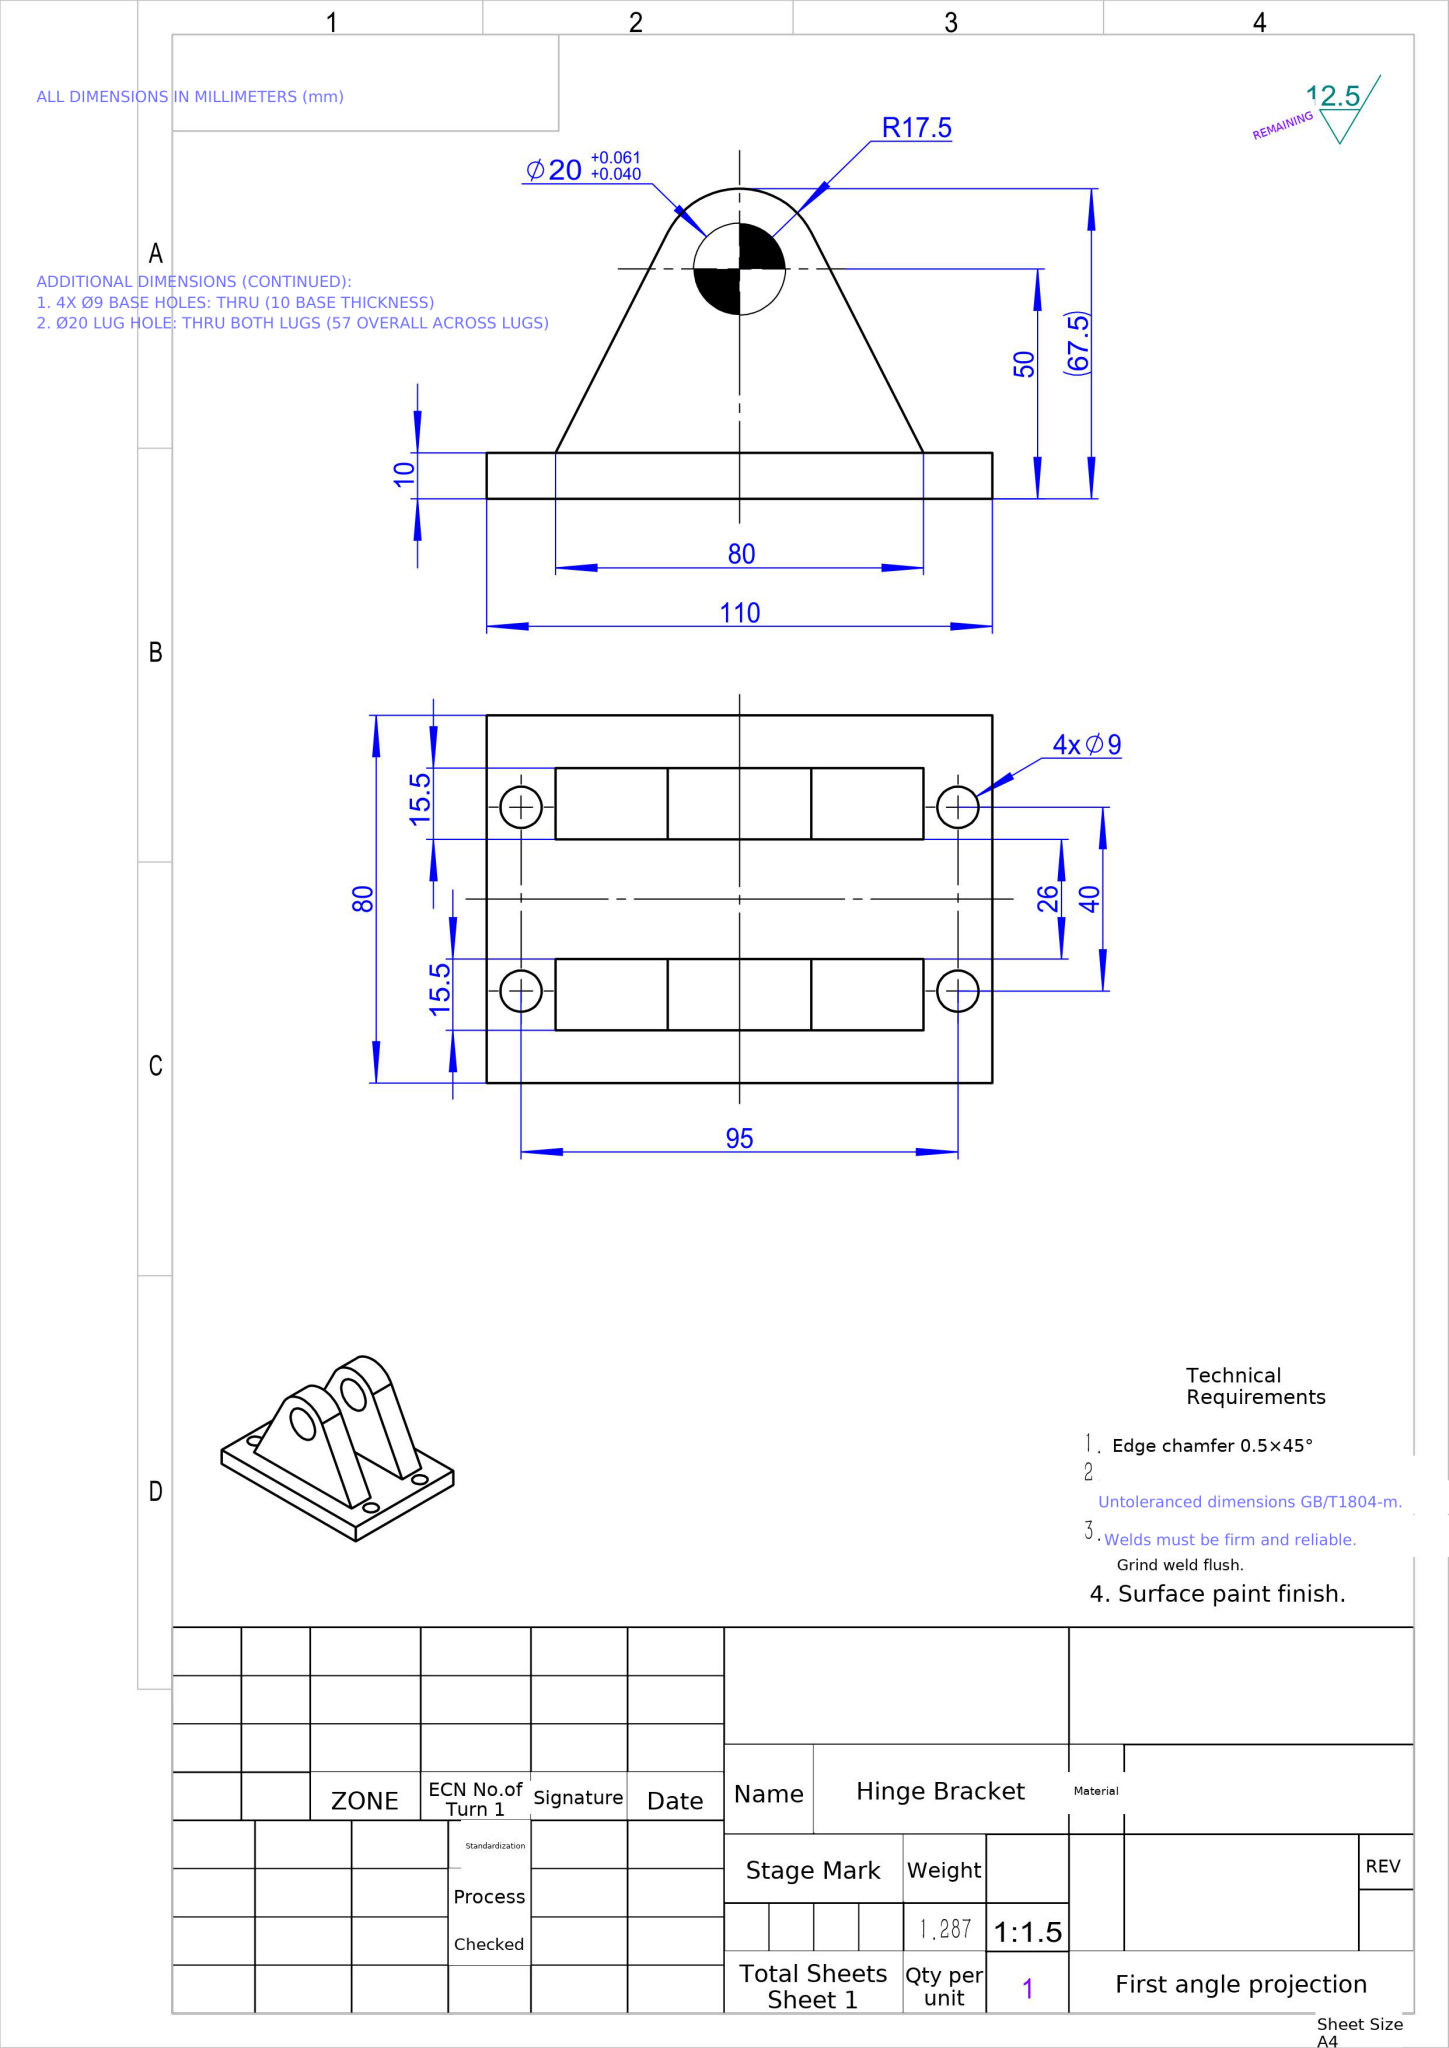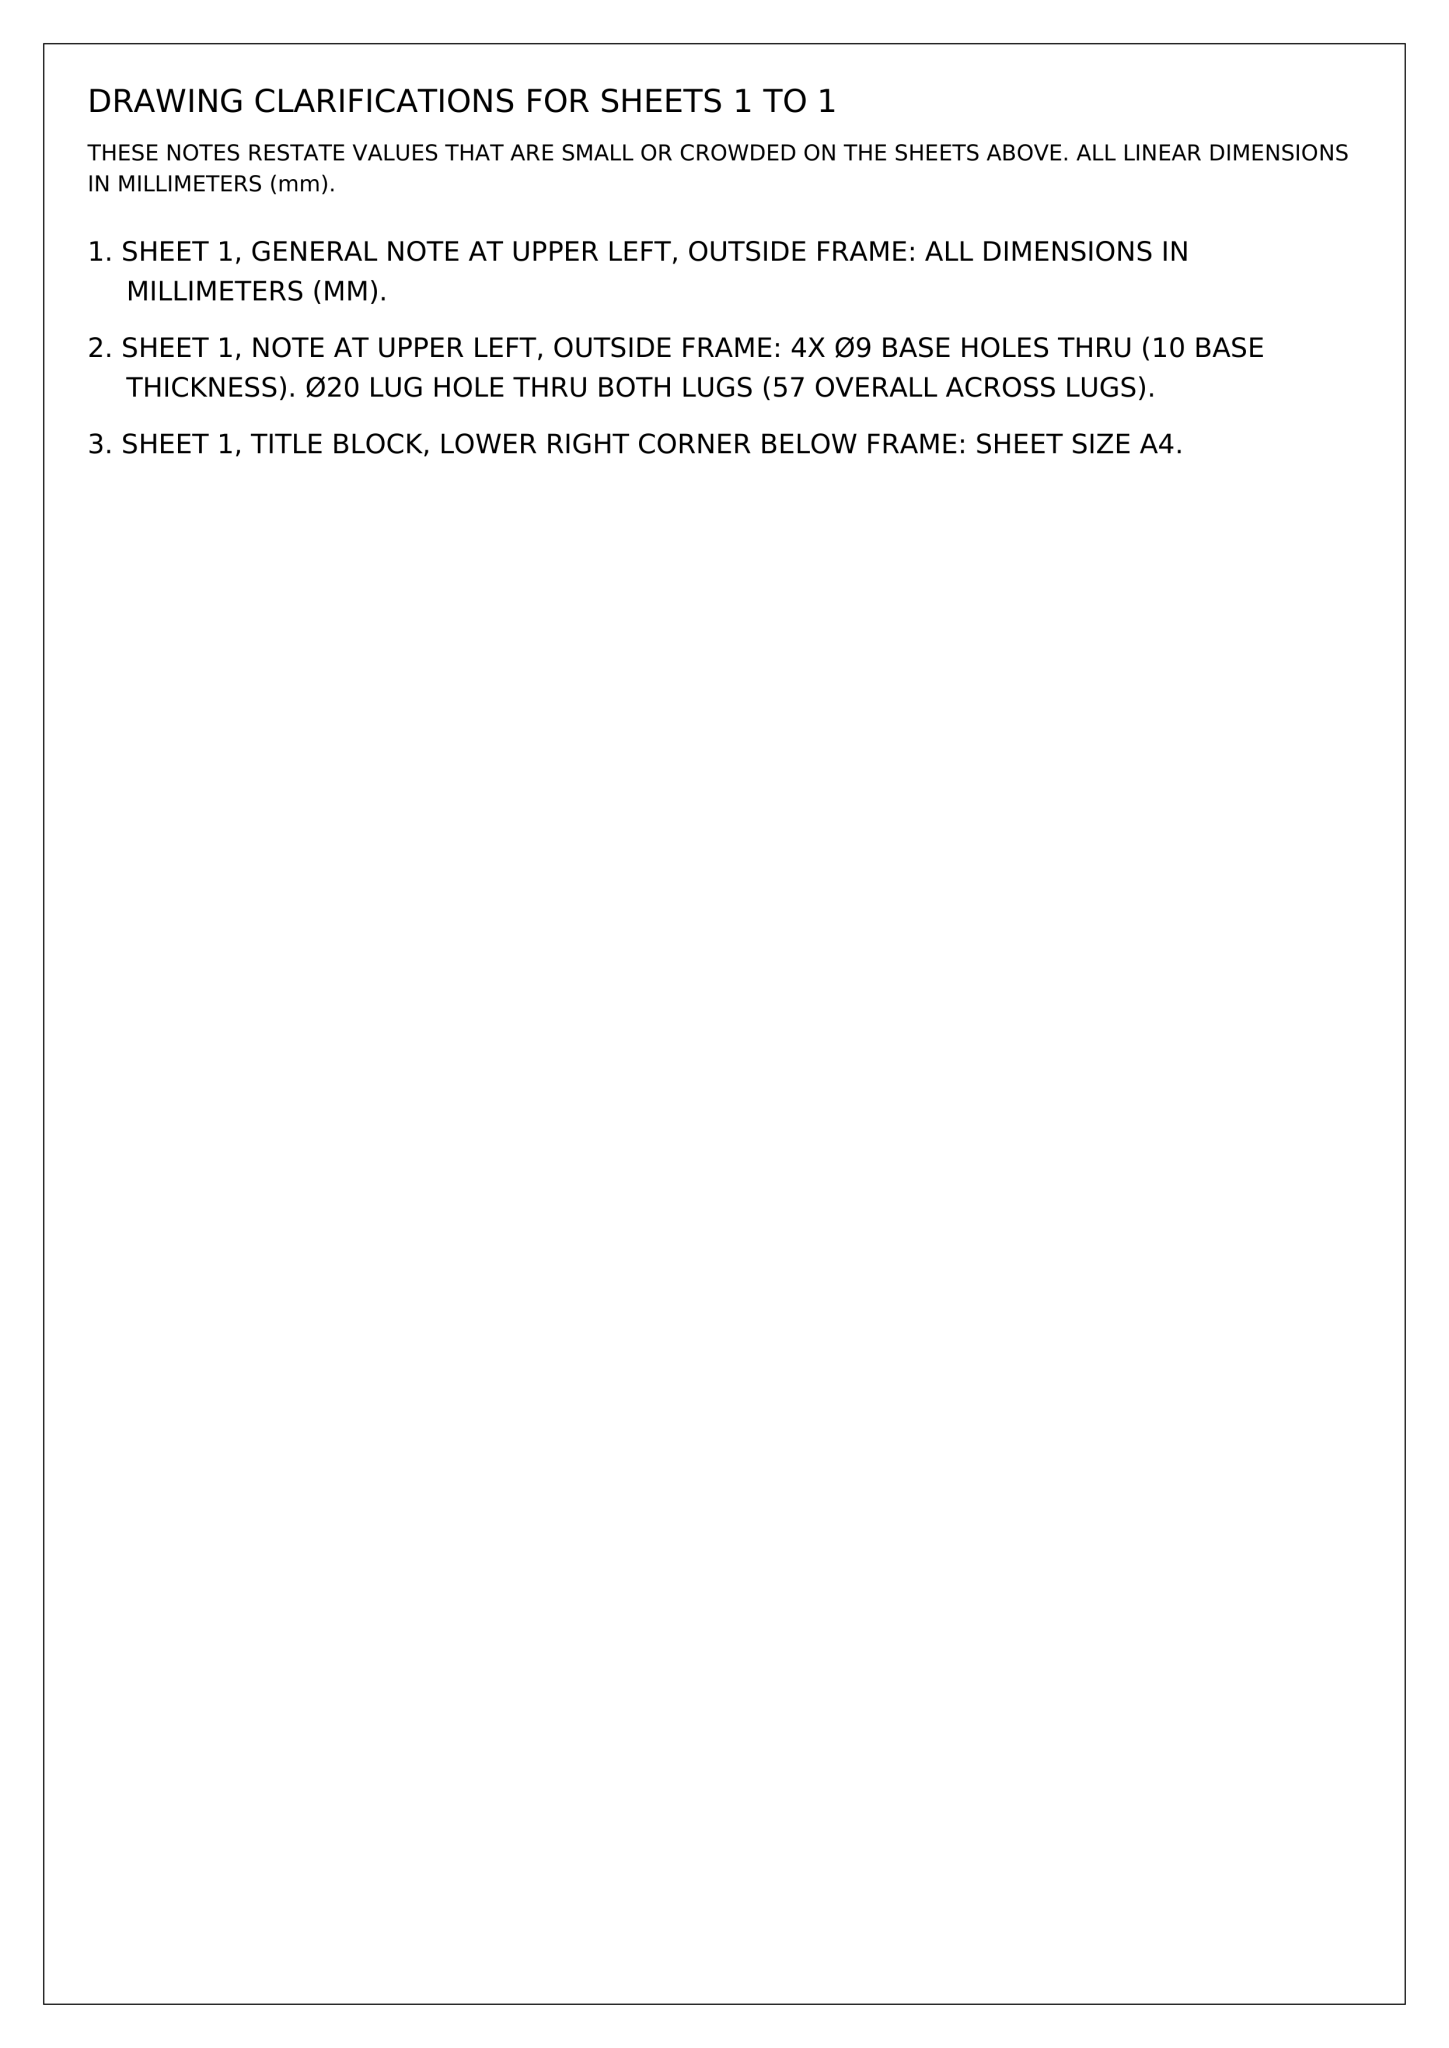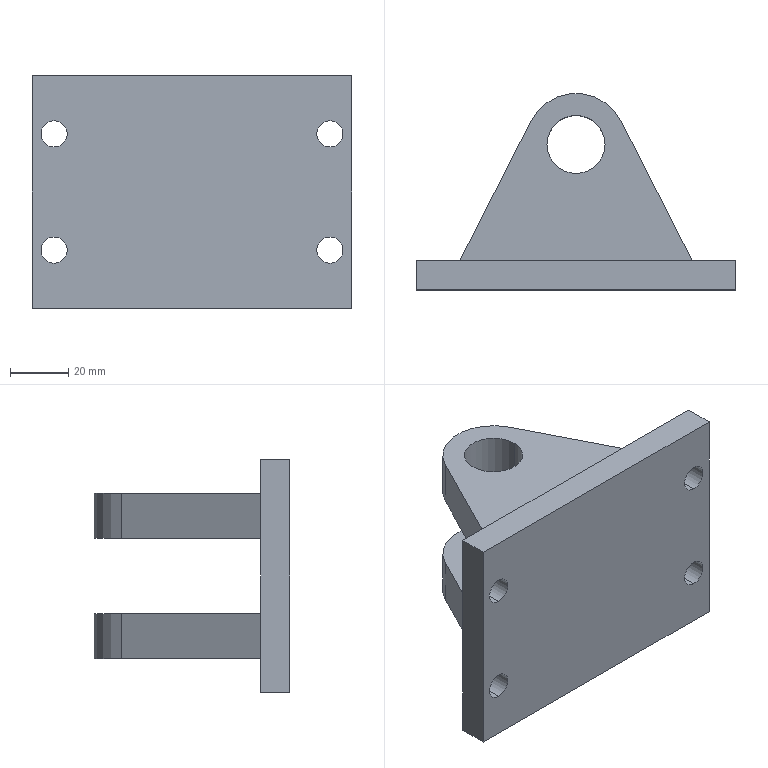Part | NX | mm | 1 solid | 28 faces | box 110 x 67.5 x 80 mm | volume 164942 mm3 | cylinder 14 | plane 14 | commonest cylinder face diameters 9 x8 20 x4 35 x2
STEP:
#1=CARTESIAN_POINT('',(10.,50.,28.5));
#2=VERTEX_POINT('',#1);
#3=CARTESIAN_POINT('',(10.,50.,13.));
#4=VERTEX_POINT('',#3);
#5=CARTESIAN_POINT('',(10.,50.,28.5));
#6=DIRECTION('',(0.,0.,-1.));
#7=VECTOR('',#6,1000.);
#8=LINE('',#5,#7);
#9=EDGE_CURVE('',#2,#4,#8,.T.);
#10=ORIENTED_EDGE('',*,*,#9,.F.);
#11=CARTESIAN_POINT('',(-10.,50.,28.5));
#12=VERTEX_POINT('',#11);
#13=CARTESIAN_POINT('',(0.,50.,28.5));
#14=DIRECTION('',(0.,0.,1.));
#15=DIRECTION('',(1.,0.,0.));
#16=AXIS2_PLACEMENT_3D('',#13,#14,#15);
#17=CIRCLE('',#16,10.);
#18=EDGE_CURVE('',#2,#12,#17,.T.);
#19=ORIENTED_EDGE('',*,*,#18,.T.);
#20=CARTESIAN_POINT('',(-10.,50.,13.));
#21=VERTEX_POINT('',#20);
#22=CARTESIAN_POINT('',(-10.,50.,28.5));
#23=DIRECTION('',(0.,0.,-1.));
#24=VECTOR('',#23,1000.);
#25=LINE('',#22,#24);
#26=EDGE_CURVE('',#12,#21,#25,.T.);
#27=ORIENTED_EDGE('',*,*,#26,.T.);
#28=CARTESIAN_POINT('',(0.,50.,13.));
#29=DIRECTION('',(0.,0.,1.));
#30=DIRECTION('',(1.,0.,0.));
#31=AXIS2_PLACEMENT_3D('',#28,#29,#30);
#32=CIRCLE('',#31,10.);
#33=EDGE_CURVE('',#4,#21,#32,.T.);
#34=ORIENTED_EDGE('',*,*,#33,.F.);
#35=EDGE_LOOP('',(#10,#19,#27,#34));
#36=FACE_OUTER_BOUND('',#35,.T.);
#37=CARTESIAN_POINT('',(0.,50.,28.5));
#38=DIRECTION('',(0.,0.,-1.));
#39=DIRECTION('',(-1.,0.,0.));
#40=AXIS2_PLACEMENT_3D('',#37,#38,#39);
#41=CYLINDRICAL_SURFACE('',#40,10.);
#42=ADVANCED_FACE('',(#36),#41,.F.);
#43=CARTESIAN_POINT('',(-15.595,57.939,13.));
#44=VERTEX_POINT('',#43);
#45=CARTESIAN_POINT('',(-40.,10.,13.));
#46=VERTEX_POINT('',#45);
#47=CARTESIAN_POINT('',(-40.,10.,13.));
#48=DIRECTION('',(-0.4537,-0.8912,0.));
#49=VECTOR('',#48,1000.);
#50=LINE('',#47,#49);
#51=EDGE_CURVE('',#44,#46,#50,.T.);
#52=ORIENTED_EDGE('',*,*,#51,.T.);
#53=CARTESIAN_POINT('',(-40.,10.,28.5));
#54=VERTEX_POINT('',#53);
#55=CARTESIAN_POINT('',(-40.,10.,28.5));
#56=DIRECTION('',(0.,0.,-1.));
#57=VECTOR('',#56,1000.);
#58=LINE('',#55,#57);
#59=EDGE_CURVE('',#54,#46,#58,.T.);
#60=ORIENTED_EDGE('',*,*,#59,.F.);
#61=CARTESIAN_POINT('',(-15.595,57.939,28.5));
#62=VERTEX_POINT('',#61);
#63=CARTESIAN_POINT('',(-40.,10.,28.5));
#64=DIRECTION('',(-0.4537,-0.8912,0.));
#65=VECTOR('',#64,1000.);
#66=LINE('',#63,#65);
#67=EDGE_CURVE('',#62,#54,#66,.T.);
#68=ORIENTED_EDGE('',*,*,#67,.F.);
#69=CARTESIAN_POINT('',(-15.595,57.939,28.5));
#70=DIRECTION('',(0.,0.,-1.));
#71=VECTOR('',#70,1000.);
#72=LINE('',#69,#71);
#73=EDGE_CURVE('',#62,#44,#72,.T.);
#74=ORIENTED_EDGE('',*,*,#73,.T.);
#75=EDGE_LOOP('',(#52,#60,#68,#74));
#76=FACE_OUTER_BOUND('',#75,.T.);
#77=CARTESIAN_POINT('',(-40.,10.,28.5));
#78=DIRECTION('',(0.8912,-0.4537,0.));
#79=DIRECTION('',(0.,0.,-1.));
#80=AXIS2_PLACEMENT_3D('',#77,#78,#79);
#81=PLANE('',#80);
#82=ADVANCED_FACE('',(#76),#81,.F.);
#83=CARTESIAN_POINT('',(15.595,57.939,13.));
#84=VERTEX_POINT('',#83);
#85=CARTESIAN_POINT('',(0.,50.,13.));
#86=DIRECTION('',(0.,0.,1.));
#87=DIRECTION('',(1.,0.,0.));
#88=AXIS2_PLACEMENT_3D('',#85,#86,#87);
#89=CIRCLE('',#88,17.5);
#90=EDGE_CURVE('',#84,#44,#89,.T.);
#91=ORIENTED_EDGE('',*,*,#90,.T.);
#92=ORIENTED_EDGE('',*,*,#73,.F.);
#93=CARTESIAN_POINT('',(15.595,57.939,28.5));
#94=VERTEX_POINT('',#93);
#95=CARTESIAN_POINT('',(0.,50.,28.5));
#96=DIRECTION('',(0.,0.,1.));
#97=DIRECTION('',(1.,0.,0.));
#98=AXIS2_PLACEMENT_3D('',#95,#96,#97);
#99=CIRCLE('',#98,17.5);
#100=EDGE_CURVE('',#94,#62,#99,.T.);
#101=ORIENTED_EDGE('',*,*,#100,.F.);
#102=CARTESIAN_POINT('',(15.595,57.939,28.5));
#103=DIRECTION('',(0.,0.,-1.));
#104=VECTOR('',#103,1000.);
#105=LINE('',#102,#104);
#106=EDGE_CURVE('',#94,#84,#105,.T.);
#107=ORIENTED_EDGE('',*,*,#106,.T.);
#108=EDGE_LOOP('',(#91,#92,#101,#107));
#109=FACE_OUTER_BOUND('',#108,.T.);
#110=CARTESIAN_POINT('',(0.,50.,28.5));
#111=DIRECTION('',(0.,0.,-1.));
#112=DIRECTION('',(-1.,0.,0.));
#113=AXIS2_PLACEMENT_3D('',#110,#111,#112);
#114=CYLINDRICAL_SURFACE('',#113,17.5);
#115=ADVANCED_FACE('',(#109),#114,.T.);
#116=CARTESIAN_POINT('',(40.,10.,13.));
#117=VERTEX_POINT('',#116);
#118=CARTESIAN_POINT('',(40.,10.,13.));
#119=DIRECTION('',(-0.4537,0.8912,0.));
#120=VECTOR('',#119,1000.);
#121=LINE('',#118,#120);
#122=EDGE_CURVE('',#117,#84,#121,.T.);
#123=ORIENTED_EDGE('',*,*,#122,.T.);
#124=ORIENTED_EDGE('',*,*,#106,.F.);
#125=CARTESIAN_POINT('',(40.,10.,28.5));
#126=VERTEX_POINT('',#125);
#127=CARTESIAN_POINT('',(40.,10.,28.5));
#128=DIRECTION('',(-0.4537,0.8912,0.));
#129=VECTOR('',#128,1000.);
#130=LINE('',#127,#129);
#131=EDGE_CURVE('',#126,#94,#130,.T.);
#132=ORIENTED_EDGE('',*,*,#131,.F.);
#133=CARTESIAN_POINT('',(40.,10.,28.5));
#134=DIRECTION('',(0.,0.,-1.));
#135=VECTOR('',#134,1000.);
#136=LINE('',#133,#135);
#137=EDGE_CURVE('',#126,#117,#136,.T.);
#138=ORIENTED_EDGE('',*,*,#137,.T.);
#139=EDGE_LOOP('',(#123,#124,#132,#138));
#140=FACE_OUTER_BOUND('',#139,.T.);
#141=CARTESIAN_POINT('',(40.,10.,28.5));
#142=DIRECTION('',(-0.8912,-0.4537,0.));
#143=DIRECTION('',(-0.4537,0.8912,0.));
#144=AXIS2_PLACEMENT_3D('',#141,#142,#143);
#145=PLANE('',#144);
#146=ADVANCED_FACE('',(#140),#145,.F.);
#147=CARTESIAN_POINT('',(0.,50.,13.));
#148=DIRECTION('',(0.,0.,1.));
#149=DIRECTION('',(1.,0.,0.));
#150=AXIS2_PLACEMENT_3D('',#147,#148,#149);
#151=CIRCLE('',#150,10.);
#152=EDGE_CURVE('',#21,#4,#151,.T.);
#153=ORIENTED_EDGE('',*,*,#152,.T.);
#154=ORIENTED_EDGE('',*,*,#33,.T.);
#155=EDGE_LOOP('',(#153,#154));
#156=FACE_BOUND('',#155,.T.);
#157=CARTESIAN_POINT('',(-40.,10.,13.));
#158=DIRECTION('',(1.,0.,0.));
#159=VECTOR('',#158,1000.);
#160=LINE('',#157,#159);
#161=EDGE_CURVE('',#46,#117,#160,.T.);
#162=ORIENTED_EDGE('',*,*,#161,.F.);
#163=ORIENTED_EDGE('',*,*,#51,.F.);
#164=ORIENTED_EDGE('',*,*,#90,.F.);
#165=ORIENTED_EDGE('',*,*,#122,.F.);
#166=EDGE_LOOP('',(#162,#163,#164,#165));
#167=FACE_OUTER_BOUND('',#166,.T.);
#168=CARTESIAN_POINT('',(0.,50.,13.));
#169=DIRECTION('',(0.,0.,1.));
#170=DIRECTION('',(1.,0.,0.));
#171=AXIS2_PLACEMENT_3D('',#168,#169,#170);
#172=PLANE('',#171);
#173=ADVANCED_FACE('',(#156,#167),#172,.F.);
#174=CARTESIAN_POINT('',(0.,50.,28.5));
#175=DIRECTION('',(0.,0.,1.));
#176=DIRECTION('',(1.,0.,0.));
#177=AXIS2_PLACEMENT_3D('',#174,#175,#176);
#178=CIRCLE('',#177,10.);
#179=EDGE_CURVE('',#12,#2,#178,.T.);
#180=ORIENTED_EDGE('',*,*,#179,.F.);
#181=ORIENTED_EDGE('',*,*,#18,.F.);
#182=EDGE_LOOP('',(#180,#181));
#183=FACE_BOUND('',#182,.T.);
#184=CARTESIAN_POINT('',(-40.,10.,28.5));
#185=DIRECTION('',(1.,0.,0.));
#186=VECTOR('',#185,1000.);
#187=LINE('',#184,#186);
#188=EDGE_CURVE('',#54,#126,#187,.T.);
#189=ORIENTED_EDGE('',*,*,#188,.T.);
#190=ORIENTED_EDGE('',*,*,#131,.T.);
#191=ORIENTED_EDGE('',*,*,#100,.T.);
#192=ORIENTED_EDGE('',*,*,#67,.T.);
#193=EDGE_LOOP('',(#189,#190,#191,#192));
#194=FACE_OUTER_BOUND('',#193,.T.);
#195=CARTESIAN_POINT('',(0.,50.,28.5));
#196=DIRECTION('',(0.,0.,1.));
#197=DIRECTION('',(1.,0.,0.));
#198=AXIS2_PLACEMENT_3D('',#195,#196,#197);
#199=PLANE('',#198);
#200=ADVANCED_FACE('',(#183,#194),#199,.T.);
#201=ORIENTED_EDGE('',*,*,#179,.T.);
#202=ORIENTED_EDGE('',*,*,#9,.T.);
#203=ORIENTED_EDGE('',*,*,#152,.F.);
#204=ORIENTED_EDGE('',*,*,#26,.F.);
#205=EDGE_LOOP('',(#201,#202,#203,#204));
#206=FACE_OUTER_BOUND('',#205,.T.);
#207=CARTESIAN_POINT('',(0.,50.,28.5));
#208=DIRECTION('',(0.,0.,-1.));
#209=DIRECTION('',(-1.,0.,0.));
#210=AXIS2_PLACEMENT_3D('',#207,#208,#209);
#211=CYLINDRICAL_SURFACE('',#210,10.);
#212=ADVANCED_FACE('',(#206),#211,.F.);
#213=CARTESIAN_POINT('',(10.,50.,-28.5));
#214=VERTEX_POINT('',#213);
#215=CARTESIAN_POINT('',(10.,50.,-13.));
#216=VERTEX_POINT('',#215);
#217=CARTESIAN_POINT('',(10.,50.,-28.5));
#218=DIRECTION('',(0.,0.,1.));
#219=VECTOR('',#218,1000.);
#220=LINE('',#217,#219);
#221=EDGE_CURVE('',#214,#216,#220,.T.);
#222=ORIENTED_EDGE('',*,*,#221,.F.);
#223=CARTESIAN_POINT('',(-10.,50.,-28.5));
#224=VERTEX_POINT('',#223);
#225=CARTESIAN_POINT('',(0.,50.,-28.5));
#226=DIRECTION('',(0.,0.,1.));
#227=DIRECTION('',(1.,0.,0.));
#228=AXIS2_PLACEMENT_3D('',#225,#226,#227);
#229=CIRCLE('',#228,10.);
#230=EDGE_CURVE('',#224,#214,#229,.T.);
#231=ORIENTED_EDGE('',*,*,#230,.F.);
#232=CARTESIAN_POINT('',(-10.,50.,-13.));
#233=VERTEX_POINT('',#232);
#234=CARTESIAN_POINT('',(-10.,50.,-28.5));
#235=DIRECTION('',(0.,0.,1.));
#236=VECTOR('',#235,1000.);
#237=LINE('',#234,#236);
#238=EDGE_CURVE('',#224,#233,#237,.T.);
#239=ORIENTED_EDGE('',*,*,#238,.T.);
#240=CARTESIAN_POINT('',(0.,50.,-13.));
#241=DIRECTION('',(0.,0.,1.));
#242=DIRECTION('',(1.,0.,0.));
#243=AXIS2_PLACEMENT_3D('',#240,#241,#242);
#244=CIRCLE('',#243,10.);
#245=EDGE_CURVE('',#233,#216,#244,.T.);
#246=ORIENTED_EDGE('',*,*,#245,.T.);
#247=EDGE_LOOP('',(#222,#231,#239,#246));
#248=FACE_OUTER_BOUND('',#247,.T.);
#249=CARTESIAN_POINT('',(0.,50.,-28.5));
#250=DIRECTION('',(0.,0.,1.));
#251=DIRECTION('',(-1.,0.,0.));
#252=AXIS2_PLACEMENT_3D('',#249,#250,#251);
#253=CYLINDRICAL_SURFACE('',#252,10.);
#254=ADVANCED_FACE('',(#248),#253,.F.);
#255=CARTESIAN_POINT('',(-15.595,57.939,-13.));
#256=VERTEX_POINT('',#255);
#257=CARTESIAN_POINT('',(-40.,10.,-13.));
#258=VERTEX_POINT('',#257);
#259=CARTESIAN_POINT('',(-40.,10.,-13.));
#260=DIRECTION('',(-0.4537,-0.8912,0.));
#261=VECTOR('',#260,1000.);
#262=LINE('',#259,#261);
#263=EDGE_CURVE('',#256,#258,#262,.T.);
#264=ORIENTED_EDGE('',*,*,#263,.F.);
#265=CARTESIAN_POINT('',(-15.595,57.939,-28.5));
#266=VERTEX_POINT('',#265);
#267=CARTESIAN_POINT('',(-15.595,57.939,-28.5));
#268=DIRECTION('',(0.,0.,1.));
#269=VECTOR('',#268,1000.);
#270=LINE('',#267,#269);
#271=EDGE_CURVE('',#266,#256,#270,.T.);
#272=ORIENTED_EDGE('',*,*,#271,.F.);
#273=CARTESIAN_POINT('',(-40.,10.,-28.5));
#274=VERTEX_POINT('',#273);
#275=CARTESIAN_POINT('',(-40.,10.,-28.5));
#276=DIRECTION('',(-0.4537,-0.8912,0.));
#277=VECTOR('',#276,1000.);
#278=LINE('',#275,#277);
#279=EDGE_CURVE('',#266,#274,#278,.T.);
#280=ORIENTED_EDGE('',*,*,#279,.T.);
#281=CARTESIAN_POINT('',(-40.,10.,-28.5));
#282=DIRECTION('',(0.,0.,1.));
#283=VECTOR('',#282,1000.);
#284=LINE('',#281,#283);
#285=EDGE_CURVE('',#274,#258,#284,.T.);
#286=ORIENTED_EDGE('',*,*,#285,.T.);
#287=EDGE_LOOP('',(#264,#272,#280,#286));
#288=FACE_OUTER_BOUND('',#287,.T.);
#289=CARTESIAN_POINT('',(-40.,10.,-28.5));
#290=DIRECTION('',(0.8912,-0.4537,0.));
#291=DIRECTION('',(0.,0.,-1.));
#292=AXIS2_PLACEMENT_3D('',#289,#290,#291);
#293=PLANE('',#292);
#294=ADVANCED_FACE('',(#288),#293,.F.);
#295=CARTESIAN_POINT('',(15.595,57.939,-13.));
#296=VERTEX_POINT('',#295);
#297=CARTESIAN_POINT('',(0.,50.,-13.));
#298=DIRECTION('',(0.,0.,1.));
#299=DIRECTION('',(1.,0.,0.));
#300=AXIS2_PLACEMENT_3D('',#297,#298,#299);
#301=CIRCLE('',#300,17.5);
#302=EDGE_CURVE('',#296,#256,#301,.T.);
#303=ORIENTED_EDGE('',*,*,#302,.F.);
#304=CARTESIAN_POINT('',(15.595,57.939,-28.5));
#305=VERTEX_POINT('',#304);
#306=CARTESIAN_POINT('',(15.595,57.939,-28.5));
#307=DIRECTION('',(0.,0.,1.));
#308=VECTOR('',#307,1000.);
#309=LINE('',#306,#308);
#310=EDGE_CURVE('',#305,#296,#309,.T.);
#311=ORIENTED_EDGE('',*,*,#310,.F.);
#312=CARTESIAN_POINT('',(0.,50.,-28.5));
#313=DIRECTION('',(0.,0.,1.));
#314=DIRECTION('',(1.,0.,0.));
#315=AXIS2_PLACEMENT_3D('',#312,#313,#314);
#316=CIRCLE('',#315,17.5);
#317=EDGE_CURVE('',#305,#266,#316,.T.);
#318=ORIENTED_EDGE('',*,*,#317,.T.);
#319=ORIENTED_EDGE('',*,*,#271,.T.);
#320=EDGE_LOOP('',(#303,#311,#318,#319));
#321=FACE_OUTER_BOUND('',#320,.T.);
#322=CARTESIAN_POINT('',(0.,50.,-28.5));
#323=DIRECTION('',(0.,0.,1.));
#324=DIRECTION('',(-1.,0.,0.));
#325=AXIS2_PLACEMENT_3D('',#322,#323,#324);
#326=CYLINDRICAL_SURFACE('',#325,17.5);
#327=ADVANCED_FACE('',(#321),#326,.T.);
#328=CARTESIAN_POINT('',(40.,10.,-13.));
#329=VERTEX_POINT('',#328);
#330=CARTESIAN_POINT('',(40.,10.,-13.));
#331=DIRECTION('',(-0.4537,0.8912,0.));
#332=VECTOR('',#331,1000.);
#333=LINE('',#330,#332);
#334=EDGE_CURVE('',#329,#296,#333,.T.);
#335=ORIENTED_EDGE('',*,*,#334,.F.);
#336=CARTESIAN_POINT('',(40.,10.,-28.5));
#337=VERTEX_POINT('',#336);
#338=CARTESIAN_POINT('',(40.,10.,-28.5));
#339=DIRECTION('',(0.,0.,1.));
#340=VECTOR('',#339,1000.);
#341=LINE('',#338,#340);
#342=EDGE_CURVE('',#337,#329,#341,.T.);
#343=ORIENTED_EDGE('',*,*,#342,.F.);
#344=CARTESIAN_POINT('',(40.,10.,-28.5));
#345=DIRECTION('',(-0.4537,0.8912,0.));
#346=VECTOR('',#345,1000.);
#347=LINE('',#344,#346);
#348=EDGE_CURVE('',#337,#305,#347,.T.);
#349=ORIENTED_EDGE('',*,*,#348,.T.);
#350=ORIENTED_EDGE('',*,*,#310,.T.);
#351=EDGE_LOOP('',(#335,#343,#349,#350));
#352=FACE_OUTER_BOUND('',#351,.T.);
#353=CARTESIAN_POINT('',(40.,10.,-28.5));
#354=DIRECTION('',(-0.8912,-0.4537,0.));
#355=DIRECTION('',(-0.4537,0.8912,0.));
#356=AXIS2_PLACEMENT_3D('',#353,#354,#355);
#357=PLANE('',#356);
#358=ADVANCED_FACE('',(#352),#357,.F.);
#359=ORIENTED_EDGE('',*,*,#245,.F.);
#360=CARTESIAN_POINT('',(0.,50.,-13.));
#361=DIRECTION('',(0.,0.,1.));
#362=DIRECTION('',(1.,0.,0.));
#363=AXIS2_PLACEMENT_3D('',#360,#361,#362);
#364=CIRCLE('',#363,10.);
#365=EDGE_CURVE('',#216,#233,#364,.T.);
#366=ORIENTED_EDGE('',*,*,#365,.F.);
#367=EDGE_LOOP('',(#359,#366));
#368=FACE_BOUND('',#367,.T.);
#369=CARTESIAN_POINT('',(-40.,10.,-13.));
#370=DIRECTION('',(1.,0.,0.));
#371=VECTOR('',#370,1000.);
#372=LINE('',#369,#371);
#373=EDGE_CURVE('',#258,#329,#372,.T.);
#374=ORIENTED_EDGE('',*,*,#373,.T.);
#375=ORIENTED_EDGE('',*,*,#334,.T.);
#376=ORIENTED_EDGE('',*,*,#302,.T.);
#377=ORIENTED_EDGE('',*,*,#263,.T.);
#378=EDGE_LOOP('',(#374,#375,#376,#377));
#379=FACE_OUTER_BOUND('',#378,.T.);
#380=CARTESIAN_POINT('',(0.,50.,-13.));
#381=DIRECTION('',(0.,0.,-1.));
#382=DIRECTION('',(0.,-1.,0.));
#383=AXIS2_PLACEMENT_3D('',#380,#381,#382);
#384=PLANE('',#383);
#385=ADVANCED_FACE('',(#368,#379),#384,.F.);
#386=ORIENTED_EDGE('',*,*,#230,.T.);
#387=CARTESIAN_POINT('',(0.,50.,-28.5));
#388=DIRECTION('',(0.,0.,1.));
#389=DIRECTION('',(1.,0.,0.));
#390=AXIS2_PLACEMENT_3D('',#387,#388,#389);
#391=CIRCLE('',#390,10.);
#392=EDGE_CURVE('',#214,#224,#391,.T.);
#393=ORIENTED_EDGE('',*,*,#392,.T.);
#394=EDGE_LOOP('',(#386,#393));
#395=FACE_BOUND('',#394,.T.);
#396=CARTESIAN_POINT('',(-40.,10.,-28.5));
#397=DIRECTION('',(1.,0.,0.));
#398=VECTOR('',#397,1000.);
#399=LINE('',#396,#398);
#400=EDGE_CURVE('',#274,#337,#399,.T.);
#401=ORIENTED_EDGE('',*,*,#400,.F.);
#402=ORIENTED_EDGE('',*,*,#279,.F.);
#403=ORIENTED_EDGE('',*,*,#317,.F.);
#404=ORIENTED_EDGE('',*,*,#348,.F.);
#405=EDGE_LOOP('',(#401,#402,#403,#404));
#406=FACE_OUTER_BOUND('',#405,.T.);
#407=CARTESIAN_POINT('',(0.,50.,-28.5));
#408=DIRECTION('',(0.,0.,-1.));
#409=DIRECTION('',(0.,-1.,0.));
#410=AXIS2_PLACEMENT_3D('',#407,#408,#409);
#411=PLANE('',#410);
#412=ADVANCED_FACE('',(#395,#406),#411,.T.);
#413=ORIENTED_EDGE('',*,*,#392,.F.);
#414=ORIENTED_EDGE('',*,*,#221,.T.);
#415=ORIENTED_EDGE('',*,*,#365,.T.);
#416=ORIENTED_EDGE('',*,*,#238,.F.);
#417=EDGE_LOOP('',(#413,#414,#415,#416));
#418=FACE_OUTER_BOUND('',#417,.T.);
#419=CARTESIAN_POINT('',(0.,50.,-28.5));
#420=DIRECTION('',(0.,0.,1.));
#421=DIRECTION('',(-1.,0.,0.));
#422=AXIS2_PLACEMENT_3D('',#419,#420,#421);
#423=CYLINDRICAL_SURFACE('',#422,10.);
#424=ADVANCED_FACE('',(#418),#423,.F.);
#425=ORIENTED_EDGE('',*,*,#59,.T.);
#426=ORIENTED_EDGE('',*,*,#161,.T.);
#427=ORIENTED_EDGE('',*,*,#137,.F.);
#428=ORIENTED_EDGE('',*,*,#188,.F.);
#429=EDGE_LOOP('',(#425,#426,#427,#428));
#430=FACE_BOUND('',#429,.T.);
#431=CARTESIAN_POINT('',(55.,10.,40.));
#432=VERTEX_POINT('',#431);
#433=CARTESIAN_POINT('',(55.,10.,-40.));
#434=VERTEX_POINT('',#433);
#435=CARTESIAN_POINT('',(55.,10.,-40.));
#436=DIRECTION('',(-0.,0.,-1.));
#437=VECTOR('',#436,1000.);
#438=LINE('',#435,#437);
#439=EDGE_CURVE('',#432,#434,#438,.T.);
#440=ORIENTED_EDGE('',*,*,#439,.T.);
#441=CARTESIAN_POINT('',(-55.,10.,-40.));
#442=VERTEX_POINT('',#441);
#443=CARTESIAN_POINT('',(-55.,10.,-40.));
#444=DIRECTION('',(-1.,0.,0.));
#445=VECTOR('',#444,1000.);
#446=LINE('',#443,#445);
#447=EDGE_CURVE('',#434,#442,#446,.T.);
#448=ORIENTED_EDGE('',*,*,#447,.T.);
#449=CARTESIAN_POINT('',(-55.,10.,40.));
#450=VERTEX_POINT('',#449);
#451=CARTESIAN_POINT('',(-55.,10.,-40.));
#452=DIRECTION('',(0.,0.,1.));
#453=VECTOR('',#452,1000.);
#454=LINE('',#451,#453);
#455=EDGE_CURVE('',#442,#450,#454,.T.);
#456=ORIENTED_EDGE('',*,*,#455,.T.);
#457=CARTESIAN_POINT('',(-55.,10.,40.));
#458=DIRECTION('',(1.,0.,0.));
#459=VECTOR('',#458,1000.);
#460=LINE('',#457,#459);
#461=EDGE_CURVE('',#450,#432,#460,.T.);
#462=ORIENTED_EDGE('',*,*,#461,.T.);
#463=EDGE_LOOP('',(#440,#448,#456,#462));
#464=FACE_OUTER_BOUND('',#463,.T.);
#465=CARTESIAN_POINT('',(-47.5,10.,24.5));
#466=VERTEX_POINT('',#465);
#467=CARTESIAN_POINT('',(-47.5,10.,15.5));
#468=VERTEX_POINT('',#467);
#469=CARTESIAN_POINT('',(-47.5,10.,20.));
#470=DIRECTION('',(0.,1.,0.));
#471=DIRECTION('',(0.,0.,-1.));
#472=AXIS2_PLACEMENT_3D('',#469,#470,#471);
#473=CIRCLE('',#472,4.5);
#474=EDGE_CURVE('',#466,#468,#473,.T.);
#475=ORIENTED_EDGE('',*,*,#474,.F.);
#476=CARTESIAN_POINT('',(-47.5,10.,20.));
#477=DIRECTION('',(0.,1.,0.));
#478=DIRECTION('',(0.,0.,-1.));
#479=AXIS2_PLACEMENT_3D('',#476,#477,#478);
#480=CIRCLE('',#479,4.5);
#481=EDGE_CURVE('',#468,#466,#480,.T.);
#482=ORIENTED_EDGE('',*,*,#481,.F.);
#483=EDGE_LOOP('',(#475,#482));
#484=FACE_BOUND('',#483,.T.);
#485=CARTESIAN_POINT('',(47.5,10.,24.5));
#486=VERTEX_POINT('',#485);
#487=CARTESIAN_POINT('',(47.5,10.,15.5));
#488=VERTEX_POINT('',#487);
#489=CARTESIAN_POINT('',(47.5,10.,20.));
#490=DIRECTION('',(0.,1.,0.));
#491=DIRECTION('',(0.,0.,1.));
#492=AXIS2_PLACEMENT_3D('',#489,#490,#491);
#493=CIRCLE('',#492,4.5);
#494=EDGE_CURVE('',#486,#488,#493,.T.);
#495=ORIENTED_EDGE('',*,*,#494,.F.);
#496=CARTESIAN_POINT('',(47.5,10.,20.));
#497=DIRECTION('',(0.,1.,0.));
#498=DIRECTION('',(0.,0.,1.));
#499=AXIS2_PLACEMENT_3D('',#496,#497,#498);
#500=CIRCLE('',#499,4.5);
#501=EDGE_CURVE('',#488,#486,#500,.T.);
#502=ORIENTED_EDGE('',*,*,#501,.F.);
#503=EDGE_LOOP('',(#495,#502));
#504=FACE_BOUND('',#503,.T.);
#505=CARTESIAN_POINT('',(47.5,10.,-15.5));
#506=VERTEX_POINT('',#505);
#507=CARTESIAN_POINT('',(47.5,10.,-24.5));
#508=VERTEX_POINT('',#507);
#509=CARTESIAN_POINT('',(47.5,10.,-20.));
#510=DIRECTION('',(0.,1.,0.));
#511=DIRECTION('',(0.,0.,-1.));
#512=AXIS2_PLACEMENT_3D('',#509,#510,#511);
#513=CIRCLE('',#512,4.5);
#514=EDGE_CURVE('',#506,#508,#513,.T.);
#515=ORIENTED_EDGE('',*,*,#514,.F.);
#516=CARTESIAN_POINT('',(47.5,10.,-20.));
#517=DIRECTION('',(0.,1.,0.));
#518=DIRECTION('',(0.,0.,-1.));
#519=AXIS2_PLACEMENT_3D('',#516,#517,#518);
#520=CIRCLE('',#519,4.5);
#521=EDGE_CURVE('',#508,#506,#520,.T.);
#522=ORIENTED_EDGE('',*,*,#521,.F.);
#523=EDGE_LOOP('',(#515,#522));
#524=FACE_BOUND('',#523,.T.);
#525=CARTESIAN_POINT('',(-47.5,10.,-15.5));
#526=VERTEX_POINT('',#525);
#527=CARTESIAN_POINT('',(-47.5,10.,-24.5));
#528=VERTEX_POINT('',#527);
#529=CARTESIAN_POINT('',(-47.5,10.,-20.));
#530=DIRECTION('',(0.,1.,0.));
#531=DIRECTION('',(0.,0.,1.));
#532=AXIS2_PLACEMENT_3D('',#529,#530,#531);
#533=CIRCLE('',#532,4.5);
#534=EDGE_CURVE('',#526,#528,#533,.T.);
#535=ORIENTED_EDGE('',*,*,#534,.F.);
#536=CARTESIAN_POINT('',(-47.5,10.,-20.));
#537=DIRECTION('',(0.,1.,0.));
#538=DIRECTION('',(0.,0.,1.));
#539=AXIS2_PLACEMENT_3D('',#536,#537,#538);
#540=CIRCLE('',#539,4.5);
#541=EDGE_CURVE('',#528,#526,#540,.T.);
#542=ORIENTED_EDGE('',*,*,#541,.F.);
#543=EDGE_LOOP('',(#535,#542));
#544=FACE_BOUND('',#543,.T.);
#545=ORIENTED_EDGE('',*,*,#373,.F.);
#546=ORIENTED_EDGE('',*,*,#285,.F.);
#547=ORIENTED_EDGE('',*,*,#400,.T.);
#548=ORIENTED_EDGE('',*,*,#342,.T.);
#549=EDGE_LOOP('',(#545,#546,#547,#548));
#550=FACE_BOUND('',#549,.T.);
#551=CARTESIAN_POINT('',(0.,10.,0.));
#552=DIRECTION('',(0.,1.,0.));
#553=DIRECTION('',(1.,0.,0.));
#554=AXIS2_PLACEMENT_3D('',#551,#552,#553);
#555=PLANE('',#554);
#556=ADVANCED_FACE('',(#430,#464,#484,#504,#524,#544,#550),#555,.T.);
#557=CARTESIAN_POINT('',(-47.5,0.,15.5));
#558=VERTEX_POINT('',#557);
#559=CARTESIAN_POINT('',(-47.5,0.,15.5));
#560=DIRECTION('',(0.,1.,0.));
#561=VECTOR('',#560,1000.);
#562=LINE('',#559,#561);
#563=EDGE_CURVE('',#558,#468,#562,.T.);
#564=ORIENTED_EDGE('',*,*,#563,.F.);
#565=CARTESIAN_POINT('',(-47.5,0.,24.5));
#566=VERTEX_POINT('',#565);
#567=CARTESIAN_POINT('',(-47.5,0.,20.));
#568=DIRECTION('',(0.,1.,0.));
#569=DIRECTION('',(0.,0.,-1.));
#570=AXIS2_PLACEMENT_3D('',#567,#568,#569);
#571=CIRCLE('',#570,4.5);
#572=EDGE_CURVE('',#566,#558,#571,.T.);
#573=ORIENTED_EDGE('',*,*,#572,.F.);
#574=CARTESIAN_POINT('',(-47.5,0.,24.5));
#575=DIRECTION('',(0.,1.,0.));
#576=VECTOR('',#575,1000.);
#577=LINE('',#574,#576);
#578=EDGE_CURVE('',#566,#466,#577,.T.);
#579=ORIENTED_EDGE('',*,*,#578,.T.);
#580=ORIENTED_EDGE('',*,*,#474,.T.);
#581=EDGE_LOOP('',(#564,#573,#579,#580));
#582=FACE_OUTER_BOUND('',#581,.T.);
#583=CARTESIAN_POINT('',(-47.5,0.,20.));
#584=DIRECTION('',(0.,1.,0.));
#585=DIRECTION('',(0.,0.,1.));
#586=AXIS2_PLACEMENT_3D('',#583,#584,#585);
#587=CYLINDRICAL_SURFACE('',#586,4.5);
#588=ADVANCED_FACE('',(#582),#587,.F.);
#589=CARTESIAN_POINT('',(47.5,0.,15.5));
#590=VERTEX_POINT('',#589);
#591=CARTESIAN_POINT('',(47.5,0.,15.5));
#592=DIRECTION('',(0.,1.,0.));
#593=VECTOR('',#592,1000.);
#594=LINE('',#591,#593);
#595=EDGE_CURVE('',#590,#488,#594,.T.);
#596=ORIENTED_EDGE('',*,*,#595,.F.);
#597=CARTESIAN_POINT('',(47.5,0.,24.5));
#598=VERTEX_POINT('',#597);
#599=CARTESIAN_POINT('',(47.5,0.,20.));
#600=DIRECTION('',(0.,1.,0.));
#601=DIRECTION('',(0.,0.,1.));
#602=AXIS2_PLACEMENT_3D('',#599,#600,#601);
#603=CIRCLE('',#602,4.5);
#604=EDGE_CURVE('',#598,#590,#603,.T.);
#605=ORIENTED_EDGE('',*,*,#604,.F.);
#606=CARTESIAN_POINT('',(47.5,0.,24.5));
#607=DIRECTION('',(0.,1.,0.));
#608=VECTOR('',#607,1000.);
#609=LINE('',#606,#608);
#610=EDGE_CURVE('',#598,#486,#609,.T.);
#611=ORIENTED_EDGE('',*,*,#610,.T.);
#612=ORIENTED_EDGE('',*,*,#494,.T.);
#613=EDGE_LOOP('',(#596,#605,#611,#612));
#614=FACE_OUTER_BOUND('',#613,.T.);
#615=CARTESIAN_POINT('',(47.5,0.,20.));
#616=DIRECTION('',(0.,1.,0.));
#617=DIRECTION('',(0.,0.,1.));
#618=AXIS2_PLACEMENT_3D('',#615,#616,#617);
#619=CYLINDRICAL_SURFACE('',#618,4.5);
#620=ADVANCED_FACE('',(#614),#619,.F.);
#621=CARTESIAN_POINT('',(47.5,0.,-24.5));
#622=VERTEX_POINT('',#621);
#623=CARTESIAN_POINT('',(47.5,0.,-24.5));
#624=DIRECTION('',(0.,1.,0.));
#625=VECTOR('',#624,1000.);
#626=LINE('',#623,#625);
#627=EDGE_CURVE('',#622,#508,#626,.T.);
#628=ORIENTED_EDGE('',*,*,#627,.F.);
#629=CARTESIAN_POINT('',(47.5,0.,-15.5));
#630=VERTEX_POINT('',#629);
#631=CARTESIAN_POINT('',(47.5,0.,-20.));
#632=DIRECTION('',(0.,1.,0.));
#633=DIRECTION('',(0.,0.,-1.));
#634=AXIS2_PLACEMENT_3D('',#631,#632,#633);
#635=CIRCLE('',#634,4.5);
#636=EDGE_CURVE('',#630,#622,#635,.T.);
#637=ORIENTED_EDGE('',*,*,#636,.F.);
#638=CARTESIAN_POINT('',(47.5,0.,-15.5));
#639=DIRECTION('',(0.,1.,0.));
#640=VECTOR('',#639,1000.);
#641=LINE('',#638,#640);
#642=EDGE_CURVE('',#630,#506,#641,.T.);
#643=ORIENTED_EDGE('',*,*,#642,.T.);
#644=ORIENTED_EDGE('',*,*,#514,.T.);
#645=EDGE_LOOP('',(#628,#637,#643,#644));
#646=FACE_OUTER_BOUND('',#645,.T.);
#647=CARTESIAN_POINT('',(47.5,0.,-20.));
#648=DIRECTION('',(0.,1.,0.));
#649=DIRECTION('',(0.,0.,1.));
#650=AXIS2_PLACEMENT_3D('',#647,#648,#649);
#651=CYLINDRICAL_SURFACE('',#650,4.5);
#652=ADVANCED_FACE('',(#646),#651,.F.);
#653=CARTESIAN_POINT('',(-47.5,0.,-24.5));
#654=VERTEX_POINT('',#653);
#655=CARTESIAN_POINT('',(-47.5,0.,-24.5));
#656=DIRECTION('',(0.,1.,0.));
#657=VECTOR('',#656,1000.);
#658=LINE('',#655,#657);
#659=EDGE_CURVE('',#654,#528,#658,.T.);
#660=ORIENTED_EDGE('',*,*,#659,.F.);
#661=CARTESIAN_POINT('',(-47.5,0.,-15.5));
#662=VERTEX_POINT('',#661);
#663=CARTESIAN_POINT('',(-47.5,0.,-20.));
#664=DIRECTION('',(0.,1.,0.));
#665=DIRECTION('',(0.,0.,1.));
#666=AXIS2_PLACEMENT_3D('',#663,#664,#665);
#667=CIRCLE('',#666,4.5);
#668=EDGE_CURVE('',#662,#654,#667,.T.);
#669=ORIENTED_EDGE('',*,*,#668,.F.);
#670=CARTESIAN_POINT('',(-47.5,0.,-15.5));
#671=DIRECTION('',(0.,1.,0.));
#672=VECTOR('',#671,1000.);
#673=LINE('',#670,#672);
#674=EDGE_CURVE('',#662,#526,#673,.T.);
#675=ORIENTED_EDGE('',*,*,#674,.T.);
#676=ORIENTED_EDGE('',*,*,#534,.T.);
#677=EDGE_LOOP('',(#660,#669,#675,#676));
#678=FACE_OUTER_BOUND('',#677,.T.);
#679=CARTESIAN_POINT('',(-47.5,0.,-20.));
#680=DIRECTION('',(0.,1.,0.));
#681=DIRECTION('',(0.,0.,1.));
#682=AXIS2_PLACEMENT_3D('',#679,#680,#681);
#683=CYLINDRICAL_SURFACE('',#682,4.5);
#684=ADVANCED_FACE('',(#678),#683,.F.);
#685=ORIENTED_EDGE('',*,*,#668,.T.);
#686=CARTESIAN_POINT('',(-47.5,0.,-20.));
#687=DIRECTION('',(0.,1.,0.));
#688=DIRECTION('',(0.,0.,1.));
#689=AXIS2_PLACEMENT_3D('',#686,#687,#688);
#690=CIRCLE('',#689,4.5);
#691=EDGE_CURVE('',#654,#662,#690,.T.);
#692=ORIENTED_EDGE('',*,*,#691,.T.);
#693=EDGE_LOOP('',(#685,#692));
#694=FACE_BOUND('',#693,.T.);
#695=ORIENTED_EDGE('',*,*,#636,.T.);
#696=CARTESIAN_POINT('',(47.5,0.,-20.));
#697=DIRECTION('',(0.,1.,0.));
#698=DIRECTION('',(0.,0.,-1.));
#699=AXIS2_PLACEMENT_3D('',#696,#697,#698);
#700=CIRCLE('',#699,4.5);
#701=EDGE_CURVE('',#622,#630,#700,.T.);
#702=ORIENTED_EDGE('',*,*,#701,.T.);
#703=EDGE_LOOP('',(#695,#702));
#704=FACE_BOUND('',#703,.T.);
#705=ORIENTED_EDGE('',*,*,#604,.T.);
#706=CARTESIAN_POINT('',(47.5,0.,20.));
#707=DIRECTION('',(0.,1.,0.));
#708=DIRECTION('',(0.,0.,1.));
#709=AXIS2_PLACEMENT_3D('',#706,#707,#708);
#710=CIRCLE('',#709,4.5);
#711=EDGE_CURVE('',#590,#598,#710,.T.);
#712=ORIENTED_EDGE('',*,*,#711,.T.);
#713=EDGE_LOOP('',(#705,#712));
#714=FACE_BOUND('',#713,.T.);
#715=ORIENTED_EDGE('',*,*,#572,.T.);
#716=CARTESIAN_POINT('',(-47.5,0.,20.));
#717=DIRECTION('',(0.,1.,0.));
#718=DIRECTION('',(0.,0.,-1.));
#719=AXIS2_PLACEMENT_3D('',#716,#717,#718);
#720=CIRCLE('',#719,4.5);
#721=EDGE_CURVE('',#558,#566,#720,.T.);
#722=ORIENTED_EDGE('',*,*,#721,.T.);
#723=EDGE_LOOP('',(#715,#722));
#724=FACE_BOUND('',#723,.T.);
#725=CARTESIAN_POINT('',(55.,0.,40.));
#726=VERTEX_POINT('',#725);
#727=CARTESIAN_POINT('',(55.,0.,-40.));
#728=VERTEX_POINT('',#727);
#729=CARTESIAN_POINT('',(55.,0.,-40.));
#730=DIRECTION('',(-0.,0.,-1.));
#731=VECTOR('',#730,1000.);
#732=LINE('',#729,#731);
#733=EDGE_CURVE('',#726,#728,#732,.T.);
#734=ORIENTED_EDGE('',*,*,#733,.F.);
#735=CARTESIAN_POINT('',(-55.,0.,40.));
#736=VERTEX_POINT('',#735);
#737=CARTESIAN_POINT('',(-55.,0.,40.));
#738=DIRECTION('',(1.,0.,0.));
#739=VECTOR('',#738,1000.);
#740=LINE('',#737,#739);
#741=EDGE_CURVE('',#736,#726,#740,.T.);
#742=ORIENTED_EDGE('',*,*,#741,.F.);
#743=CARTESIAN_POINT('',(-55.,0.,-40.));
#744=VERTEX_POINT('',#743);
#745=CARTESIAN_POINT('',(-55.,0.,-40.));
#746=DIRECTION('',(0.,0.,1.));
#747=VECTOR('',#746,1000.);
#748=LINE('',#745,#747);
#749=EDGE_CURVE('',#744,#736,#748,.T.);
#750=ORIENTED_EDGE('',*,*,#749,.F.);
#751=CARTESIAN_POINT('',(-55.,0.,-40.));
#752=DIRECTION('',(-1.,0.,0.));
#753=VECTOR('',#752,1000.);
#754=LINE('',#751,#753);
#755=EDGE_CURVE('',#728,#744,#754,.T.);
#756=ORIENTED_EDGE('',*,*,#755,.F.);
#757=EDGE_LOOP('',(#734,#742,#750,#756));
#758=FACE_OUTER_BOUND('',#757,.T.);
#759=CARTESIAN_POINT('',(0.,0.,0.));
#760=DIRECTION('',(0.,1.,0.));
#761=DIRECTION('',(1.,0.,0.));
#762=AXIS2_PLACEMENT_3D('',#759,#760,#761);
#763=PLANE('',#762);
#764=ADVANCED_FACE('',(#694,#704,#714,#724,#758),#763,.F.);
#765=ORIENTED_EDGE('',*,*,#741,.T.);
#766=CARTESIAN_POINT('',(55.,10.,40.));
#767=DIRECTION('',(0.,-1.,0.));
#768=VECTOR('',#767,1000.);
#769=LINE('',#766,#768);
#770=EDGE_CURVE('',#432,#726,#769,.T.);
#771=ORIENTED_EDGE('',*,*,#770,.F.);
#772=ORIENTED_EDGE('',*,*,#461,.F.);
#773=CARTESIAN_POINT('',(-55.,10.,40.));
#774=DIRECTION('',(0.,-1.,0.));
#775=VECTOR('',#774,1000.);
#776=LINE('',#773,#775);
#777=EDGE_CURVE('',#450,#736,#776,.T.);
#778=ORIENTED_EDGE('',*,*,#777,.T.);
#779=EDGE_LOOP('',(#765,#771,#772,#778));
#780=FACE_OUTER_BOUND('',#779,.T.);
#781=CARTESIAN_POINT('',(-55.,10.,40.));
#782=DIRECTION('',(0.,0.,-1.));
#783=DIRECTION('',(0.,-1.,0.));
#784=AXIS2_PLACEMENT_3D('',#781,#782,#783);
#785=PLANE('',#784);
#786=ADVANCED_FACE('',(#780),#785,.F.);
#787=ORIENTED_EDGE('',*,*,#749,.T.);
#788=ORIENTED_EDGE('',*,*,#777,.F.);
#789=ORIENTED_EDGE('',*,*,#455,.F.);
#790=CARTESIAN_POINT('',(-55.,10.,-40.));
#791=DIRECTION('',(0.,-1.,0.));
#792=VECTOR('',#791,1000.);
#793=LINE('',#790,#792);
#794=EDGE_CURVE('',#442,#744,#793,.T.);
#795=ORIENTED_EDGE('',*,*,#794,.T.);
#796=EDGE_LOOP('',(#787,#788,#789,#795));
#797=FACE_OUTER_BOUND('',#796,.T.);
#798=CARTESIAN_POINT('',(-55.,10.,-40.));
#799=DIRECTION('',(1.,0.,-0.));
#800=DIRECTION('',(-0.,0.,-1.));
#801=AXIS2_PLACEMENT_3D('',#798,#799,#800);
#802=PLANE('',#801);
#803=ADVANCED_FACE('',(#797),#802,.F.);
#804=ORIENTED_EDGE('',*,*,#755,.T.);
#805=ORIENTED_EDGE('',*,*,#794,.F.);
#806=ORIENTED_EDGE('',*,*,#447,.F.);
#807=CARTESIAN_POINT('',(55.,10.,-40.));
#808=DIRECTION('',(0.,-1.,0.));
#809=VECTOR('',#808,1000.);
#810=LINE('',#807,#809);
#811=EDGE_CURVE('',#434,#728,#810,.T.);
#812=ORIENTED_EDGE('',*,*,#811,.T.);
#813=EDGE_LOOP('',(#804,#805,#806,#812));
#814=FACE_OUTER_BOUND('',#813,.T.);
#815=CARTESIAN_POINT('',(-55.,10.,-40.));
#816=DIRECTION('',(0.,0.,1.));
#817=DIRECTION('',(1.,0.,0.));
#818=AXIS2_PLACEMENT_3D('',#815,#816,#817);
#819=PLANE('',#818);
#820=ADVANCED_FACE('',(#814),#819,.F.);
#821=ORIENTED_EDGE('',*,*,#733,.T.);
#822=ORIENTED_EDGE('',*,*,#811,.F.);
#823=ORIENTED_EDGE('',*,*,#439,.F.);
#824=ORIENTED_EDGE('',*,*,#770,.T.);
#825=EDGE_LOOP('',(#821,#822,#823,#824));
#826=FACE_OUTER_BOUND('',#825,.T.);
#827=CARTESIAN_POINT('',(55.,10.,-40.));
#828=DIRECTION('',(-1.,0.,0.));
#829=DIRECTION('',(0.,1.,0.));
#830=AXIS2_PLACEMENT_3D('',#827,#828,#829);
#831=PLANE('',#830);
#832=ADVANCED_FACE('',(#826),#831,.F.);
#833=ORIENTED_EDGE('',*,*,#691,.F.);
#834=ORIENTED_EDGE('',*,*,#659,.T.);
#835=ORIENTED_EDGE('',*,*,#541,.T.);
#836=ORIENTED_EDGE('',*,*,#674,.F.);
#837=EDGE_LOOP('',(#833,#834,#835,#836));
#838=FACE_OUTER_BOUND('',#837,.T.);
#839=CARTESIAN_POINT('',(-47.5,0.,-20.));
#840=DIRECTION('',(0.,1.,0.));
#841=DIRECTION('',(0.,0.,1.));
#842=AXIS2_PLACEMENT_3D('',#839,#840,#841);
#843=CYLINDRICAL_SURFACE('',#842,4.5);
#844=ADVANCED_FACE('',(#838),#843,.F.);
#845=ORIENTED_EDGE('',*,*,#701,.F.);
#846=ORIENTED_EDGE('',*,*,#627,.T.);
#847=ORIENTED_EDGE('',*,*,#521,.T.);
#848=ORIENTED_EDGE('',*,*,#642,.F.);
#849=EDGE_LOOP('',(#845,#846,#847,#848));
#850=FACE_OUTER_BOUND('',#849,.T.);
#851=CARTESIAN_POINT('',(47.5,0.,-20.));
#852=DIRECTION('',(0.,1.,0.));
#853=DIRECTION('',(0.,0.,1.));
#854=AXIS2_PLACEMENT_3D('',#851,#852,#853);
#855=CYLINDRICAL_SURFACE('',#854,4.5);
#856=ADVANCED_FACE('',(#850),#855,.F.);
#857=ORIENTED_EDGE('',*,*,#711,.F.);
#858=ORIENTED_EDGE('',*,*,#595,.T.);
#859=ORIENTED_EDGE('',*,*,#501,.T.);
#860=ORIENTED_EDGE('',*,*,#610,.F.);
#861=EDGE_LOOP('',(#857,#858,#859,#860));
#862=FACE_OUTER_BOUND('',#861,.T.);
#863=CARTESIAN_POINT('',(47.5,0.,20.));
#864=DIRECTION('',(0.,1.,0.));
#865=DIRECTION('',(0.,0.,1.));
#866=AXIS2_PLACEMENT_3D('',#863,#864,#865);
#867=CYLINDRICAL_SURFACE('',#866,4.5);
#868=ADVANCED_FACE('',(#862),#867,.F.);
#869=ORIENTED_EDGE('',*,*,#721,.F.);
#870=ORIENTED_EDGE('',*,*,#563,.T.);
#871=ORIENTED_EDGE('',*,*,#481,.T.);
#872=ORIENTED_EDGE('',*,*,#578,.F.);
#873=EDGE_LOOP('',(#869,#870,#871,#872));
#874=FACE_OUTER_BOUND('',#873,.T.);
#875=CARTESIAN_POINT('',(-47.5,0.,20.));
#876=DIRECTION('',(0.,1.,0.));
#877=DIRECTION('',(0.,0.,1.));
#878=AXIS2_PLACEMENT_3D('',#875,#876,#877);
#879=CYLINDRICAL_SURFACE('',#878,4.5);
#880=ADVANCED_FACE('',(#874),#879,.F.);
#881=CLOSED_SHELL('',(#42,#82,#115,#146,#173,#200,#212,#254,#294,#327,#358,#385,#412,#424,#556,#588,#620,#652,#684,#764,#786,#803,#820,#832,#844,#856,#868,#880));
#882=MANIFOLD_SOLID_BREP('',#881);
#883=CARTESIAN_POINT('',(0.,0.,0.));
#884=DIRECTION('',(0.,0.,1.));
#885=DIRECTION('',(1.,0.,0.));
#886=AXIS2_PLACEMENT_3D('',#883,#884,#885);
#887=(LENGTH_UNIT()NAMED_UNIT(*)SI_UNIT(.MILLI.,.METRE.));
#888=UNCERTAINTY_MEASURE_WITH_UNIT(LENGTH_MEASURE(0.00001),#887,'','');
#889=(NAMED_UNIT(*)PLANE_ANGLE_UNIT()SI_UNIT($,.RADIAN.));
#890=(NAMED_UNIT(*)SI_UNIT($,.STERADIAN.)SOLID_ANGLE_UNIT());
#891=(GEOMETRIC_REPRESENTATION_CONTEXT(3)GLOBAL_UNCERTAINTY_ASSIGNED_CONTEXT((#888))GLOBAL_UNIT_ASSIGNED_CONTEXT((#887,#889,#890))REPRESENTATION_CONTEXT('',''));
#892=ADVANCED_BREP_SHAPE_REPRESENTATION('',(#882,#886),#891);
#893=COLOUR_RGB('',0.7922,0.8196,0.9333);
#894=FILL_AREA_STYLE_COLOUR('',#893);
#895=FILL_AREA_STYLE('',(#894));
#896=SURFACE_STYLE_FILL_AREA(#895);
#897=SURFACE_SIDE_STYLE('',(#896));
#898=SURFACE_STYLE_USAGE(.BOTH.,#897);
#899=PRESENTATION_STYLE_ASSIGNMENT((#898));
#900=STYLED_ITEM('',(#899),#882);
#901=PRESENTATION_LAYER_ASSIGNMENT('','',(#900));
#902=(LENGTH_UNIT()NAMED_UNIT(*)SI_UNIT(.MILLI.,.METRE.));
#903=UNCERTAINTY_MEASURE_WITH_UNIT(LENGTH_MEASURE(0.00001),#902,'','');
#904=(NAMED_UNIT(*)PLANE_ANGLE_UNIT()SI_UNIT($,.RADIAN.));
#905=(NAMED_UNIT(*)SI_UNIT($,.STERADIAN.)SOLID_ANGLE_UNIT());
#906=(GEOMETRIC_REPRESENTATION_CONTEXT(3)GLOBAL_UNCERTAINTY_ASSIGNED_CONTEXT((#903))GLOBAL_UNIT_ASSIGNED_CONTEXT((#902,#904,#905))REPRESENTATION_CONTEXT('',''));
#907=MECHANICAL_DESIGN_GEOMETRIC_PRESENTATION_REPRESENTATION('',(#900),#906);